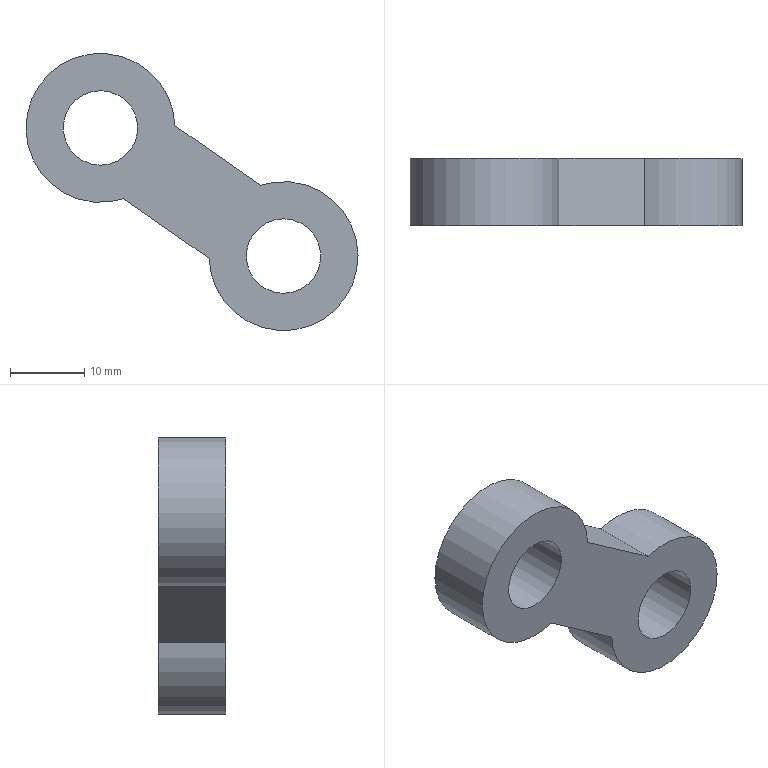Component | NX | CONNECTING_ROD_2_2 | 1 solid | 8 faces | box 44.57 x 9 x 37.21 mm | volume 5459 mm3 | cylinder 4 | plane 4 | commonest cylinder face diameters 20 x2 10 x2
STEP:
#1=CARTESIAN_POINT('',(0.,0.,0.));
#2=DIRECTION('',(0.,0.,1.));
#3=DIRECTION('',(1.,0.,0.));
#4=AXIS2_PLACEMENT_3D('',#1,#2,#3);
#5=CARTESIAN_POINT('',(-59.406,-25.005,107.534));
#6=VERTEX_POINT('',#5);
#7=CARTESIAN_POINT('',(-66.289,-25.005,97.704));
#8=VERTEX_POINT('',#7);
#9=CARTESIAN_POINT('',(-69.401,-25.005,107.207));
#10=DIRECTION('',(0.,-1.,0.));
#11=DIRECTION('',(0.8192,0.,-0.5736));
#12=AXIS2_PLACEMENT_3D('',#9,#10,#11);
#13=CIRCLE('',#12,10.);
#14=CARTESIAN_POINT('',(-69.401,-34.005,107.207));
#15=DIRECTION('',(0.,1.,0.));
#16=DIRECTION('',(-0.8192,0.,0.5736));
#17=AXIS2_PLACEMENT_3D('',#14,#15,#16);
#18=CYLINDRICAL_SURFACE('',#17,10.);
#19=CARTESIAN_POINT('',(9.425,9.));
#20=DIRECTION('',(-1.,0.));
#21=VECTOR('',#20,1.);
#22=LINE('',#19,#21);
#23=(GEOMETRIC_REPRESENTATION_CONTEXT(2)PARAMETRIC_REPRESENTATION_CONTEXT()REPRESENTATION_CONTEXT('',''));
#24=DEFINITIONAL_REPRESENTATION('',(#22),#23);
#25=PCURVE('',#18,#24);
#26=CARTESIAN_POINT('',(-69.401,-25.005,107.207));
#27=DIRECTION('',(0.,-1.,0.));
#28=DIRECTION('',(0.8192,0.,-0.5736));
#29=AXIS2_PLACEMENT_3D('',#26,#27,#28);
#30=PLANE('',#29);
#31=CARTESIAN_POINT('',(0.,0.));
#32=DIRECTION('',(1.,0.));
#33=AXIS2_PLACEMENT_2D('',#31,#32);
#34=CIRCLE('',#33,10.);
#35=(GEOMETRIC_REPRESENTATION_CONTEXT(2)PARAMETRIC_REPRESENTATION_CONTEXT()REPRESENTATION_CONTEXT('',''));
#36=DEFINITIONAL_REPRESENTATION('',(#34),#35);
#37=PCURVE('',#30,#36);
#38=SURFACE_CURVE('',#13,(#25,#37),.PCURVE_S1.);
#39=EDGE_CURVE('',#6,#8,#38,.T.);
#40=ORIENTED_EDGE('',*,*,#39,.T.);
#41=CARTESIAN_POINT('',(-66.289,-34.005,97.704));
#42=VERTEX_POINT('',#41);
#43=CARTESIAN_POINT('',(-66.289,-34.005,97.704));
#44=DIRECTION('',(0.,1.,0.));
#45=VECTOR('',#44,1.);
#46=LINE('',#43,#45);
#47=CARTESIAN_POINT('',(3.785,0.));
#48=DIRECTION('',(0.,1.));
#49=VECTOR('',#48,1.);
#50=LINE('',#47,#49);
#51=(GEOMETRIC_REPRESENTATION_CONTEXT(2)PARAMETRIC_REPRESENTATION_CONTEXT()REPRESENTATION_CONTEXT('',''));
#52=DEFINITIONAL_REPRESENTATION('',(#50),#51);
#53=PCURVE('',#18,#52);
#54=CARTESIAN_POINT('',(-66.289,-34.005,97.704));
#55=DIRECTION('',(0.5736,0.,0.8192));
#56=DIRECTION('',(0.,-1.,0.));
#57=AXIS2_PLACEMENT_3D('',#54,#55,#56);
#58=PLANE('',#57);
#59=CARTESIAN_POINT('',(0.,0.));
#60=DIRECTION('',(-1.,0.));
#61=VECTOR('',#60,1.);
#62=LINE('',#59,#61);
#63=(GEOMETRIC_REPRESENTATION_CONTEXT(2)PARAMETRIC_REPRESENTATION_CONTEXT()REPRESENTATION_CONTEXT('',''));
#64=DEFINITIONAL_REPRESENTATION('',(#62),#63);
#65=PCURVE('',#58,#64);
#66=SURFACE_CURVE('',#46,(#53,#65),.PCURVE_S1.);
#67=EDGE_CURVE('',#42,#8,#66,.T.);
#68=ORIENTED_EDGE('',*,*,#67,.F.);
#69=CARTESIAN_POINT('',(-59.406,-34.005,107.534));
#70=VERTEX_POINT('',#69);
#71=CARTESIAN_POINT('',(-69.401,-34.005,107.207));
#72=DIRECTION('',(0.,-1.,0.));
#73=DIRECTION('',(0.8192,0.,-0.5736));
#74=AXIS2_PLACEMENT_3D('',#71,#72,#73);
#75=CIRCLE('',#74,10.);
#76=CARTESIAN_POINT('',(9.425,0.));
#77=DIRECTION('',(-1.,0.));
#78=VECTOR('',#77,1.);
#79=LINE('',#76,#78);
#80=(GEOMETRIC_REPRESENTATION_CONTEXT(2)PARAMETRIC_REPRESENTATION_CONTEXT()REPRESENTATION_CONTEXT('',''));
#81=DEFINITIONAL_REPRESENTATION('',(#79),#80);
#82=PCURVE('',#18,#81);
#83=CARTESIAN_POINT('',(-69.401,-34.005,107.207));
#84=DIRECTION('',(0.,-1.,0.));
#85=DIRECTION('',(0.8192,0.,-0.5736));
#86=AXIS2_PLACEMENT_3D('',#83,#84,#85);
#87=PLANE('',#86);
#88=CARTESIAN_POINT('',(0.,0.));
#89=DIRECTION('',(1.,0.));
#90=AXIS2_PLACEMENT_2D('',#88,#89);
#91=CIRCLE('',#90,10.);
#92=(GEOMETRIC_REPRESENTATION_CONTEXT(2)PARAMETRIC_REPRESENTATION_CONTEXT()REPRESENTATION_CONTEXT('',''));
#93=DEFINITIONAL_REPRESENTATION('',(#91),#92);
#94=PCURVE('',#87,#93);
#95=SURFACE_CURVE('',#75,(#82,#94),.PCURVE_S1.);
#96=EDGE_CURVE('',#70,#42,#95,.T.);
#97=ORIENTED_EDGE('',*,*,#96,.F.);
#98=CARTESIAN_POINT('',(-59.406,-34.005,107.534));
#99=DIRECTION('',(0.,1.,0.));
#100=VECTOR('',#99,1.);
#101=LINE('',#98,#100);
#102=CARTESIAN_POINT('',(8.781,0.));
#103=DIRECTION('',(0.,1.));
#104=VECTOR('',#103,1.);
#105=LINE('',#102,#104);
#106=(GEOMETRIC_REPRESENTATION_CONTEXT(2)PARAMETRIC_REPRESENTATION_CONTEXT()REPRESENTATION_CONTEXT('',''));
#107=DEFINITIONAL_REPRESENTATION('',(#105),#106);
#108=PCURVE('',#18,#107);
#109=CARTESIAN_POINT('',(-47.938,-34.005,99.504));
#110=DIRECTION('',(-0.5736,0.,-0.8192));
#111=DIRECTION('',(0.,1.,0.));
#112=AXIS2_PLACEMENT_3D('',#109,#110,#111);
#113=PLANE('',#112);
#114=CARTESIAN_POINT('',(0.,-14.));
#115=DIRECTION('',(1.,0.));
#116=VECTOR('',#115,1.);
#117=LINE('',#114,#116);
#118=(GEOMETRIC_REPRESENTATION_CONTEXT(2)PARAMETRIC_REPRESENTATION_CONTEXT()REPRESENTATION_CONTEXT('',''));
#119=DEFINITIONAL_REPRESENTATION('',(#117),#118);
#120=PCURVE('',#113,#119);
#121=SURFACE_CURVE('',#101,(#108,#120),.PCURVE_S1.);
#122=EDGE_CURVE('',#70,#6,#121,.T.);
#123=ORIENTED_EDGE('',*,*,#122,.T.);
#124=EDGE_LOOP('',(#40,#68,#97,#123));
#125=FACE_BOUND('',#124,.T.);
#126=ADVANCED_FACE('',(#125),#18,.T.);
#127=CARTESIAN_POINT('',(-54.821,-25.005,89.674));
#128=VERTEX_POINT('',#127);
#129=CARTESIAN_POINT('',(-66.289,-25.005,97.704));
#130=DIRECTION('',(0.8192,0.,-0.5736));
#131=VECTOR('',#130,1.);
#132=LINE('',#129,#131);
#133=CARTESIAN_POINT('',(-9.,0.));
#134=DIRECTION('',(0.,1.));
#135=VECTOR('',#134,1.);
#136=LINE('',#133,#135);
#137=(GEOMETRIC_REPRESENTATION_CONTEXT(2)PARAMETRIC_REPRESENTATION_CONTEXT()REPRESENTATION_CONTEXT('',''));
#138=DEFINITIONAL_REPRESENTATION('',(#136),#137);
#139=PCURVE('',#58,#138);
#140=CARTESIAN_POINT('',(8.,-6.));
#141=DIRECTION('',(1.,0.));
#142=VECTOR('',#141,1.);
#143=LINE('',#140,#142);
#144=(GEOMETRIC_REPRESENTATION_CONTEXT(2)PARAMETRIC_REPRESENTATION_CONTEXT()REPRESENTATION_CONTEXT('',''));
#145=DEFINITIONAL_REPRESENTATION('',(#143),#144);
#146=PCURVE('',#30,#145);
#147=SURFACE_CURVE('',#132,(#139,#146),.PCURVE_S1.);
#148=EDGE_CURVE('',#8,#128,#147,.T.);
#149=ORIENTED_EDGE('',*,*,#148,.T.);
#150=CARTESIAN_POINT('',(-54.821,-34.005,89.674));
#151=VERTEX_POINT('',#150);
#152=CARTESIAN_POINT('',(-54.821,-34.005,89.674));
#153=DIRECTION('',(0.,1.,0.));
#154=VECTOR('',#153,1.);
#155=LINE('',#152,#154);
#156=CARTESIAN_POINT('',(0.,14.));
#157=DIRECTION('',(-1.,0.));
#158=VECTOR('',#157,1.);
#159=LINE('',#156,#158);
#160=(GEOMETRIC_REPRESENTATION_CONTEXT(2)PARAMETRIC_REPRESENTATION_CONTEXT()REPRESENTATION_CONTEXT('',''));
#161=DEFINITIONAL_REPRESENTATION('',(#159),#160);
#162=PCURVE('',#58,#161);
#163=CARTESIAN_POINT('',(-44.827,-34.005,90.));
#164=DIRECTION('',(0.,1.,0.));
#165=DIRECTION('',(-0.8192,0.,0.5736));
#166=AXIS2_PLACEMENT_3D('',#163,#164,#165);
#167=CYLINDRICAL_SURFACE('',#166,10.);
#168=CARTESIAN_POINT('',(5.64,0.));
#169=DIRECTION('',(0.,1.));
#170=VECTOR('',#169,1.);
#171=LINE('',#168,#170);
#172=(GEOMETRIC_REPRESENTATION_CONTEXT(2)PARAMETRIC_REPRESENTATION_CONTEXT()REPRESENTATION_CONTEXT('',''));
#173=DEFINITIONAL_REPRESENTATION('',(#171),#172);
#174=PCURVE('',#167,#173);
#175=SURFACE_CURVE('',#155,(#162,#174),.PCURVE_S1.);
#176=EDGE_CURVE('',#151,#128,#175,.T.);
#177=ORIENTED_EDGE('',*,*,#176,.F.);
#178=CARTESIAN_POINT('',(-66.289,-34.005,97.704));
#179=DIRECTION('',(0.8192,0.,-0.5736));
#180=VECTOR('',#179,1.);
#181=LINE('',#178,#180);
#182=CARTESIAN_POINT('',(0.,0.));
#183=DIRECTION('',(0.,1.));
#184=VECTOR('',#183,1.);
#185=LINE('',#182,#184);
#186=(GEOMETRIC_REPRESENTATION_CONTEXT(2)PARAMETRIC_REPRESENTATION_CONTEXT()REPRESENTATION_CONTEXT('',''));
#187=DEFINITIONAL_REPRESENTATION('',(#185),#186);
#188=PCURVE('',#58,#187);
#189=CARTESIAN_POINT('',(8.,-6.));
#190=DIRECTION('',(1.,0.));
#191=VECTOR('',#190,1.);
#192=LINE('',#189,#191);
#193=(GEOMETRIC_REPRESENTATION_CONTEXT(2)PARAMETRIC_REPRESENTATION_CONTEXT()REPRESENTATION_CONTEXT('',''));
#194=DEFINITIONAL_REPRESENTATION('',(#192),#193);
#195=PCURVE('',#87,#194);
#196=SURFACE_CURVE('',#181,(#188,#195),.PCURVE_S1.);
#197=EDGE_CURVE('',#42,#151,#196,.T.);
#198=ORIENTED_EDGE('',*,*,#197,.F.);
#199=ORIENTED_EDGE('',*,*,#67,.T.);
#200=EDGE_LOOP('',(#149,#177,#198,#199));
#201=FACE_BOUND('',#200,.T.);
#202=ADVANCED_FACE('',(#201),#58,.F.);
#203=CARTESIAN_POINT('',(-47.938,-25.005,99.504));
#204=VERTEX_POINT('',#203);
#205=CARTESIAN_POINT('',(-44.827,-25.005,90.));
#206=DIRECTION('',(0.,-1.,0.));
#207=DIRECTION('',(0.8192,0.,-0.5736));
#208=AXIS2_PLACEMENT_3D('',#205,#206,#207);
#209=CIRCLE('',#208,10.);
#210=CARTESIAN_POINT('',(9.425,9.));
#211=DIRECTION('',(-1.,0.));
#212=VECTOR('',#211,1.);
#213=LINE('',#210,#212);
#214=(GEOMETRIC_REPRESENTATION_CONTEXT(2)PARAMETRIC_REPRESENTATION_CONTEXT()REPRESENTATION_CONTEXT('',''));
#215=DEFINITIONAL_REPRESENTATION('',(#213),#214);
#216=PCURVE('',#167,#215);
#217=CARTESIAN_POINT('',(30.,0.));
#218=DIRECTION('',(1.,0.));
#219=AXIS2_PLACEMENT_2D('',#217,#218);
#220=CIRCLE('',#219,10.);
#221=(GEOMETRIC_REPRESENTATION_CONTEXT(2)PARAMETRIC_REPRESENTATION_CONTEXT()REPRESENTATION_CONTEXT('',''));
#222=DEFINITIONAL_REPRESENTATION('',(#220),#221);
#223=PCURVE('',#30,#222);
#224=SURFACE_CURVE('',#209,(#216,#223),.PCURVE_S1.);
#225=EDGE_CURVE('',#128,#204,#224,.T.);
#226=ORIENTED_EDGE('',*,*,#225,.T.);
#227=CARTESIAN_POINT('',(-47.938,-34.005,99.504));
#228=VERTEX_POINT('',#227);
#229=CARTESIAN_POINT('',(-47.938,-34.005,99.504));
#230=DIRECTION('',(0.,1.,0.));
#231=VECTOR('',#230,1.);
#232=LINE('',#229,#231);
#233=CARTESIAN_POINT('',(0.6435,0.));
#234=DIRECTION('',(0.,1.));
#235=VECTOR('',#234,1.);
#236=LINE('',#233,#235);
#237=(GEOMETRIC_REPRESENTATION_CONTEXT(2)PARAMETRIC_REPRESENTATION_CONTEXT()REPRESENTATION_CONTEXT('',''));
#238=DEFINITIONAL_REPRESENTATION('',(#236),#237);
#239=PCURVE('',#167,#238);
#240=CARTESIAN_POINT('',(0.,0.));
#241=DIRECTION('',(1.,0.));
#242=VECTOR('',#241,1.);
#243=LINE('',#240,#242);
#244=(GEOMETRIC_REPRESENTATION_CONTEXT(2)PARAMETRIC_REPRESENTATION_CONTEXT()REPRESENTATION_CONTEXT('',''));
#245=DEFINITIONAL_REPRESENTATION('',(#243),#244);
#246=PCURVE('',#113,#245);
#247=SURFACE_CURVE('',#232,(#239,#246),.PCURVE_S1.);
#248=EDGE_CURVE('',#228,#204,#247,.T.);
#249=ORIENTED_EDGE('',*,*,#248,.F.);
#250=CARTESIAN_POINT('',(-44.827,-34.005,90.));
#251=DIRECTION('',(0.,-1.,0.));
#252=DIRECTION('',(0.8192,0.,-0.5736));
#253=AXIS2_PLACEMENT_3D('',#250,#251,#252);
#254=CIRCLE('',#253,10.);
#255=CARTESIAN_POINT('',(9.425,0.));
#256=DIRECTION('',(-1.,0.));
#257=VECTOR('',#256,1.);
#258=LINE('',#255,#257);
#259=(GEOMETRIC_REPRESENTATION_CONTEXT(2)PARAMETRIC_REPRESENTATION_CONTEXT()REPRESENTATION_CONTEXT('',''));
#260=DEFINITIONAL_REPRESENTATION('',(#258),#259);
#261=PCURVE('',#167,#260);
#262=CARTESIAN_POINT('',(30.,0.));
#263=DIRECTION('',(1.,0.));
#264=AXIS2_PLACEMENT_2D('',#262,#263);
#265=CIRCLE('',#264,10.);
#266=(GEOMETRIC_REPRESENTATION_CONTEXT(2)PARAMETRIC_REPRESENTATION_CONTEXT()REPRESENTATION_CONTEXT('',''));
#267=DEFINITIONAL_REPRESENTATION('',(#265),#266);
#268=PCURVE('',#87,#267);
#269=SURFACE_CURVE('',#254,(#261,#268),.PCURVE_S1.);
#270=EDGE_CURVE('',#151,#228,#269,.T.);
#271=ORIENTED_EDGE('',*,*,#270,.F.);
#272=ORIENTED_EDGE('',*,*,#176,.T.);
#273=EDGE_LOOP('',(#226,#249,#271,#272));
#274=FACE_BOUND('',#273,.T.);
#275=ADVANCED_FACE('',(#274),#167,.T.);
#276=CARTESIAN_POINT('',(-65.305,-34.005,104.339));
#277=VERTEX_POINT('',#276);
#278=CARTESIAN_POINT('',(-69.401,-34.005,107.207));
#279=DIRECTION('',(0.,-1.,0.));
#280=DIRECTION('',(0.8192,0.,-0.5736));
#281=AXIS2_PLACEMENT_3D('',#278,#279,#280);
#282=CIRCLE('',#281,5.);
#283=CARTESIAN_POINT('',(-69.401,-34.005,107.207));
#284=DIRECTION('',(0.,1.,0.));
#285=DIRECTION('',(-0.8192,0.,0.5736));
#286=AXIS2_PLACEMENT_3D('',#283,#284,#285);
#287=CYLINDRICAL_SURFACE('',#286,5.);
#288=CARTESIAN_POINT('',(9.425,0.));
#289=DIRECTION('',(-1.,0.));
#290=VECTOR('',#289,1.);
#291=LINE('',#288,#290);
#292=(GEOMETRIC_REPRESENTATION_CONTEXT(2)PARAMETRIC_REPRESENTATION_CONTEXT()REPRESENTATION_CONTEXT('',''));
#293=DEFINITIONAL_REPRESENTATION('',(#291),#292);
#294=PCURVE('',#287,#293);
#295=CARTESIAN_POINT('',(0.,0.));
#296=DIRECTION('',(1.,0.));
#297=AXIS2_PLACEMENT_2D('',#295,#296);
#298=CIRCLE('',#297,5.);
#299=(GEOMETRIC_REPRESENTATION_CONTEXT(2)PARAMETRIC_REPRESENTATION_CONTEXT()REPRESENTATION_CONTEXT('',''));
#300=DEFINITIONAL_REPRESENTATION('',(#298),#299);
#301=PCURVE('',#87,#300);
#302=SURFACE_CURVE('',#282,(#294,#301),.PCURVE_S1.);
#303=EDGE_CURVE('',#277,#277,#302,.T.);
#304=ORIENTED_EDGE('',*,*,#303,.F.);
#305=CARTESIAN_POINT('',(-65.305,-25.005,104.339));
#306=VERTEX_POINT('',#305);
#307=CARTESIAN_POINT('',(-65.305,-34.005,104.339));
#308=CARTESIAN_POINT('',(-65.305,-25.005,104.339));
#309=B_SPLINE_CURVE_WITH_KNOTS('',1,(#307,#308),.UNSPECIFIED.,.F.,.F.,(2,2),(0.,9.),.PIECEWISE_BEZIER_KNOTS.);
#310=CARTESIAN_POINT('',(9.425,0.));
#311=DIRECTION('',(0.,1.));
#312=VECTOR('',#311,1.);
#313=LINE('',#310,#312);
#314=(GEOMETRIC_REPRESENTATION_CONTEXT(2)PARAMETRIC_REPRESENTATION_CONTEXT()REPRESENTATION_CONTEXT('',''));
#315=DEFINITIONAL_REPRESENTATION('',(#313),#314);
#316=PCURVE('',#287,#315);
#317=CARTESIAN_POINT('',(3.142,0.));
#318=DIRECTION('',(0.,1.));
#319=VECTOR('',#318,1.);
#320=LINE('',#317,#319);
#321=(GEOMETRIC_REPRESENTATION_CONTEXT(2)PARAMETRIC_REPRESENTATION_CONTEXT()REPRESENTATION_CONTEXT('',''));
#322=DEFINITIONAL_REPRESENTATION('',(#320),#321);
#323=PCURVE('',#287,#322);
#324=SEAM_CURVE('',#309,(#316,#323),.PCURVE_S1.);
#325=EDGE_CURVE('',#277,#306,#324,.T.);
#326=ORIENTED_EDGE('',*,*,#325,.T.);
#327=CARTESIAN_POINT('',(-69.401,-25.005,107.207));
#328=DIRECTION('',(0.,-1.,0.));
#329=DIRECTION('',(0.8192,0.,-0.5736));
#330=AXIS2_PLACEMENT_3D('',#327,#328,#329);
#331=CIRCLE('',#330,5.);
#332=CARTESIAN_POINT('',(9.425,9.));
#333=DIRECTION('',(-1.,0.));
#334=VECTOR('',#333,1.);
#335=LINE('',#332,#334);
#336=(GEOMETRIC_REPRESENTATION_CONTEXT(2)PARAMETRIC_REPRESENTATION_CONTEXT()REPRESENTATION_CONTEXT('',''));
#337=DEFINITIONAL_REPRESENTATION('',(#335),#336);
#338=PCURVE('',#287,#337);
#339=CARTESIAN_POINT('',(0.,0.));
#340=DIRECTION('',(1.,0.));
#341=AXIS2_PLACEMENT_2D('',#339,#340);
#342=CIRCLE('',#341,5.);
#343=(GEOMETRIC_REPRESENTATION_CONTEXT(2)PARAMETRIC_REPRESENTATION_CONTEXT()REPRESENTATION_CONTEXT('',''));
#344=DEFINITIONAL_REPRESENTATION('',(#342),#343);
#345=PCURVE('',#30,#344);
#346=SURFACE_CURVE('',#331,(#338,#345),.PCURVE_S1.);
#347=EDGE_CURVE('',#306,#306,#346,.T.);
#348=ORIENTED_EDGE('',*,*,#347,.T.);
#349=ORIENTED_EDGE('',*,*,#325,.F.);
#350=EDGE_LOOP('',(#304,#326,#348,#349));
#351=FACE_BOUND('',#350,.F.);
#352=ADVANCED_FACE('',(#351),#287,.F.);
#353=CARTESIAN_POINT('',(-47.938,-25.005,99.504));
#354=DIRECTION('',(-0.8192,0.,0.5736));
#355=VECTOR('',#354,1.);
#356=LINE('',#353,#355);
#357=CARTESIAN_POINT('',(9.,0.));
#358=DIRECTION('',(0.,-1.));
#359=VECTOR('',#358,1.);
#360=LINE('',#357,#359);
#361=(GEOMETRIC_REPRESENTATION_CONTEXT(2)PARAMETRIC_REPRESENTATION_CONTEXT()REPRESENTATION_CONTEXT('',''));
#362=DEFINITIONAL_REPRESENTATION('',(#360),#361);
#363=PCURVE('',#113,#362);
#364=CARTESIAN_POINT('',(22.,6.));
#365=DIRECTION('',(-1.,0.));
#366=VECTOR('',#365,1.);
#367=LINE('',#364,#366);
#368=(GEOMETRIC_REPRESENTATION_CONTEXT(2)PARAMETRIC_REPRESENTATION_CONTEXT()REPRESENTATION_CONTEXT('',''));
#369=DEFINITIONAL_REPRESENTATION('',(#367),#368);
#370=PCURVE('',#30,#369);
#371=SURFACE_CURVE('',#356,(#363,#370),.PCURVE_S1.);
#372=EDGE_CURVE('',#204,#6,#371,.T.);
#373=ORIENTED_EDGE('',*,*,#372,.T.);
#374=ORIENTED_EDGE('',*,*,#122,.F.);
#375=CARTESIAN_POINT('',(-47.938,-34.005,99.504));
#376=DIRECTION('',(-0.8192,0.,0.5736));
#377=VECTOR('',#376,1.);
#378=LINE('',#375,#377);
#379=CARTESIAN_POINT('',(0.,0.));
#380=DIRECTION('',(0.,-1.));
#381=VECTOR('',#380,1.);
#382=LINE('',#379,#381);
#383=(GEOMETRIC_REPRESENTATION_CONTEXT(2)PARAMETRIC_REPRESENTATION_CONTEXT()REPRESENTATION_CONTEXT('',''));
#384=DEFINITIONAL_REPRESENTATION('',(#382),#383);
#385=PCURVE('',#113,#384);
#386=CARTESIAN_POINT('',(22.,6.));
#387=DIRECTION('',(-1.,0.));
#388=VECTOR('',#387,1.);
#389=LINE('',#386,#388);
#390=(GEOMETRIC_REPRESENTATION_CONTEXT(2)PARAMETRIC_REPRESENTATION_CONTEXT()REPRESENTATION_CONTEXT('',''));
#391=DEFINITIONAL_REPRESENTATION('',(#389),#390);
#392=PCURVE('',#87,#391);
#393=SURFACE_CURVE('',#378,(#385,#392),.PCURVE_S1.);
#394=EDGE_CURVE('',#228,#70,#393,.T.);
#395=ORIENTED_EDGE('',*,*,#394,.F.);
#396=ORIENTED_EDGE('',*,*,#248,.T.);
#397=EDGE_LOOP('',(#373,#374,#395,#396));
#398=FACE_BOUND('',#397,.T.);
#399=ADVANCED_FACE('',(#398),#113,.F.);
#400=CARTESIAN_POINT('',(-40.731,-34.005,87.132));
#401=VERTEX_POINT('',#400);
#402=CARTESIAN_POINT('',(-44.827,-34.005,90.));
#403=DIRECTION('',(0.,-1.,0.));
#404=DIRECTION('',(0.8192,0.,-0.5736));
#405=AXIS2_PLACEMENT_3D('',#402,#403,#404);
#406=CIRCLE('',#405,5.);
#407=CARTESIAN_POINT('',(-44.827,-34.005,90.));
#408=DIRECTION('',(0.,1.,0.));
#409=DIRECTION('',(-0.8192,0.,0.5736));
#410=AXIS2_PLACEMENT_3D('',#407,#408,#409);
#411=CYLINDRICAL_SURFACE('',#410,5.);
#412=CARTESIAN_POINT('',(9.425,0.));
#413=DIRECTION('',(-1.,0.));
#414=VECTOR('',#413,1.);
#415=LINE('',#412,#414);
#416=(GEOMETRIC_REPRESENTATION_CONTEXT(2)PARAMETRIC_REPRESENTATION_CONTEXT()REPRESENTATION_CONTEXT('',''));
#417=DEFINITIONAL_REPRESENTATION('',(#415),#416);
#418=PCURVE('',#411,#417);
#419=CARTESIAN_POINT('',(30.,0.));
#420=DIRECTION('',(1.,0.));
#421=AXIS2_PLACEMENT_2D('',#419,#420);
#422=CIRCLE('',#421,5.);
#423=(GEOMETRIC_REPRESENTATION_CONTEXT(2)PARAMETRIC_REPRESENTATION_CONTEXT()REPRESENTATION_CONTEXT('',''));
#424=DEFINITIONAL_REPRESENTATION('',(#422),#423);
#425=PCURVE('',#87,#424);
#426=SURFACE_CURVE('',#406,(#418,#425),.PCURVE_S1.);
#427=EDGE_CURVE('',#401,#401,#426,.T.);
#428=ORIENTED_EDGE('',*,*,#427,.F.);
#429=CARTESIAN_POINT('',(-40.731,-25.005,87.132));
#430=VERTEX_POINT('',#429);
#431=CARTESIAN_POINT('',(-40.731,-34.005,87.132));
#432=CARTESIAN_POINT('',(-40.731,-25.005,87.132));
#433=B_SPLINE_CURVE_WITH_KNOTS('',1,(#431,#432),.UNSPECIFIED.,.F.,.F.,(2,2),(0.,9.),.PIECEWISE_BEZIER_KNOTS.);
#434=CARTESIAN_POINT('',(9.425,0.));
#435=DIRECTION('',(0.,1.));
#436=VECTOR('',#435,1.);
#437=LINE('',#434,#436);
#438=(GEOMETRIC_REPRESENTATION_CONTEXT(2)PARAMETRIC_REPRESENTATION_CONTEXT()REPRESENTATION_CONTEXT('',''));
#439=DEFINITIONAL_REPRESENTATION('',(#437),#438);
#440=PCURVE('',#411,#439);
#441=CARTESIAN_POINT('',(3.142,0.));
#442=DIRECTION('',(0.,1.));
#443=VECTOR('',#442,1.);
#444=LINE('',#441,#443);
#445=(GEOMETRIC_REPRESENTATION_CONTEXT(2)PARAMETRIC_REPRESENTATION_CONTEXT()REPRESENTATION_CONTEXT('',''));
#446=DEFINITIONAL_REPRESENTATION('',(#444),#445);
#447=PCURVE('',#411,#446);
#448=SEAM_CURVE('',#433,(#440,#447),.PCURVE_S1.);
#449=EDGE_CURVE('',#401,#430,#448,.T.);
#450=ORIENTED_EDGE('',*,*,#449,.T.);
#451=CARTESIAN_POINT('',(-44.827,-25.005,90.));
#452=DIRECTION('',(0.,-1.,0.));
#453=DIRECTION('',(0.8192,0.,-0.5736));
#454=AXIS2_PLACEMENT_3D('',#451,#452,#453);
#455=CIRCLE('',#454,5.);
#456=CARTESIAN_POINT('',(9.425,9.));
#457=DIRECTION('',(-1.,0.));
#458=VECTOR('',#457,1.);
#459=LINE('',#456,#458);
#460=(GEOMETRIC_REPRESENTATION_CONTEXT(2)PARAMETRIC_REPRESENTATION_CONTEXT()REPRESENTATION_CONTEXT('',''));
#461=DEFINITIONAL_REPRESENTATION('',(#459),#460);
#462=PCURVE('',#411,#461);
#463=CARTESIAN_POINT('',(30.,0.));
#464=DIRECTION('',(1.,0.));
#465=AXIS2_PLACEMENT_2D('',#463,#464);
#466=CIRCLE('',#465,5.);
#467=(GEOMETRIC_REPRESENTATION_CONTEXT(2)PARAMETRIC_REPRESENTATION_CONTEXT()REPRESENTATION_CONTEXT('',''));
#468=DEFINITIONAL_REPRESENTATION('',(#466),#467);
#469=PCURVE('',#30,#468);
#470=SURFACE_CURVE('',#455,(#462,#469),.PCURVE_S1.);
#471=EDGE_CURVE('',#430,#430,#470,.T.);
#472=ORIENTED_EDGE('',*,*,#471,.T.);
#473=ORIENTED_EDGE('',*,*,#449,.F.);
#474=EDGE_LOOP('',(#428,#450,#472,#473));
#475=FACE_BOUND('',#474,.F.);
#476=ADVANCED_FACE('',(#475),#411,.F.);
#477=ORIENTED_EDGE('',*,*,#96,.T.);
#478=ORIENTED_EDGE('',*,*,#197,.T.);
#479=ORIENTED_EDGE('',*,*,#270,.T.);
#480=ORIENTED_EDGE('',*,*,#394,.T.);
#481=EDGE_LOOP('',(#477,#478,#479,#480));
#482=FACE_BOUND('',#481,.T.);
#483=ORIENTED_EDGE('',*,*,#303,.F.);
#484=EDGE_LOOP('',(#483));
#485=FACE_BOUND('',#484,.T.);
#486=ORIENTED_EDGE('',*,*,#427,.F.);
#487=EDGE_LOOP('',(#486));
#488=FACE_BOUND('',#487,.T.);
#489=ADVANCED_FACE('',(#482,#485,#488),#87,.T.);
#490=ORIENTED_EDGE('',*,*,#39,.F.);
#491=ORIENTED_EDGE('',*,*,#372,.F.);
#492=ORIENTED_EDGE('',*,*,#225,.F.);
#493=ORIENTED_EDGE('',*,*,#148,.F.);
#494=EDGE_LOOP('',(#490,#491,#492,#493));
#495=FACE_BOUND('',#494,.T.);
#496=ORIENTED_EDGE('',*,*,#347,.T.);
#497=EDGE_LOOP('',(#496));
#498=FACE_BOUND('',#497,.T.);
#499=ORIENTED_EDGE('',*,*,#471,.T.);
#500=EDGE_LOOP('',(#499));
#501=FACE_BOUND('',#500,.T.);
#502=ADVANCED_FACE('',(#495,#498,#501),#30,.F.);
#503=CLOSED_SHELL('',(#126,#202,#275,#352,#399,#476,#489,#502));
#504=MANIFOLD_SOLID_BREP('',#503);
#505=(LENGTH_UNIT()NAMED_UNIT(*)SI_UNIT(.MILLI.,.METRE.));
#506=UNCERTAINTY_MEASURE_WITH_UNIT(LENGTH_MEASURE(0.000002),#505,'','');
#507=(NAMED_UNIT(*)PLANE_ANGLE_UNIT()SI_UNIT($,.RADIAN.));
#508=(NAMED_UNIT(*)SI_UNIT($,.STERADIAN.)SOLID_ANGLE_UNIT());
#509=(GEOMETRIC_REPRESENTATION_CONTEXT(3)GLOBAL_UNCERTAINTY_ASSIGNED_CONTEXT((#506))GLOBAL_UNIT_ASSIGNED_CONTEXT((#505,#507,#508))REPRESENTATION_CONTEXT('',''));
#510=ADVANCED_BREP_SHAPE_REPRESENTATION('',(#4,#504),#509);